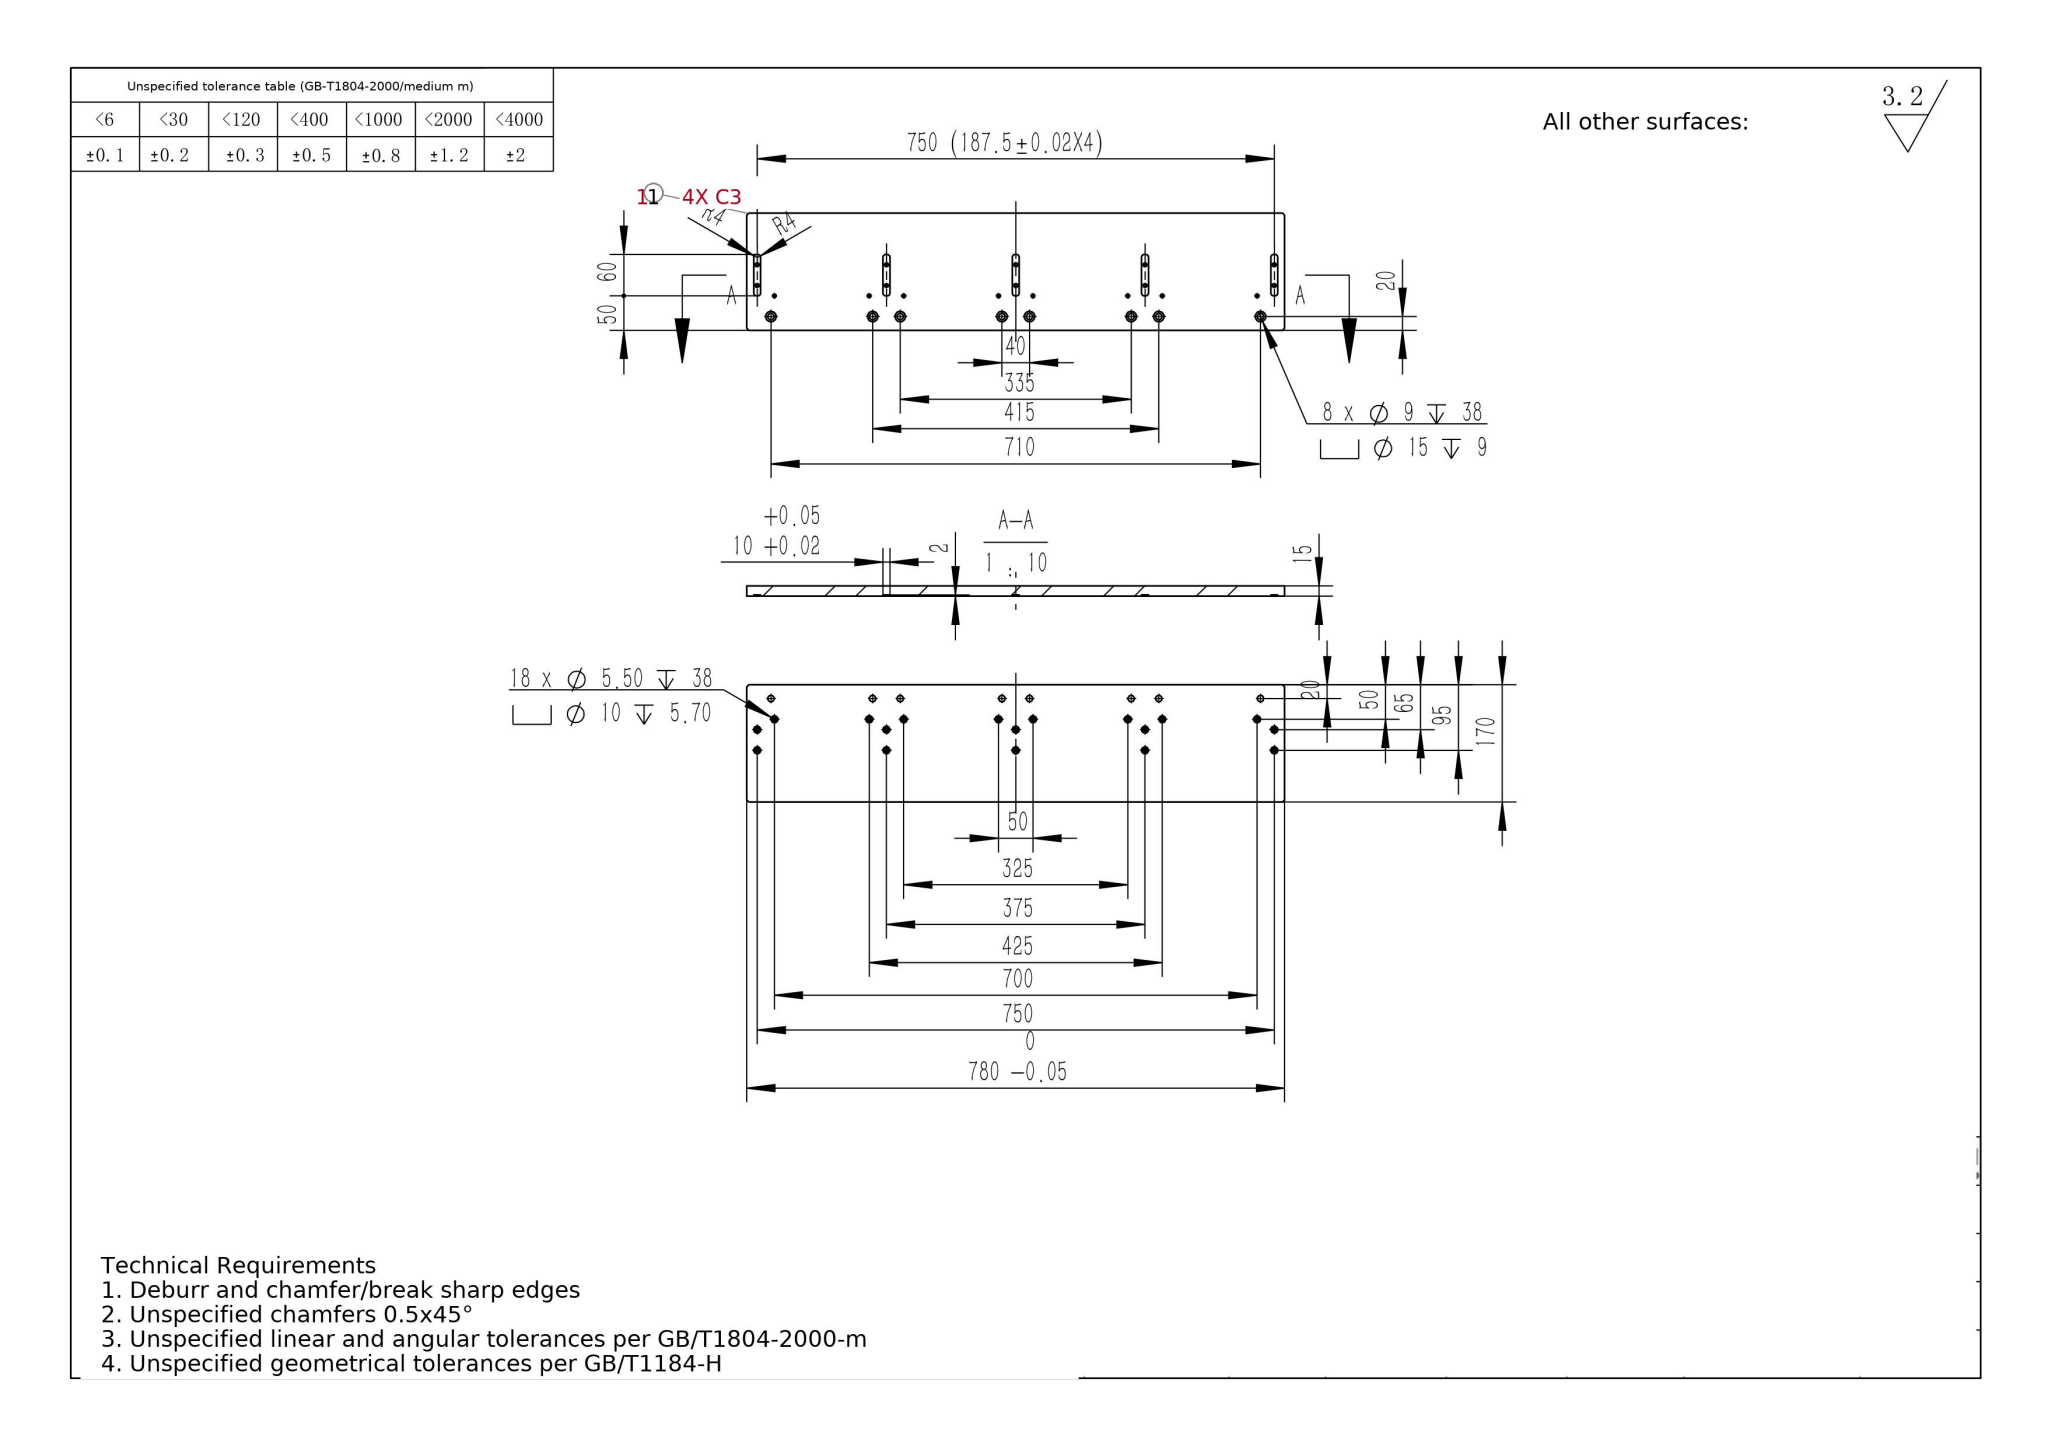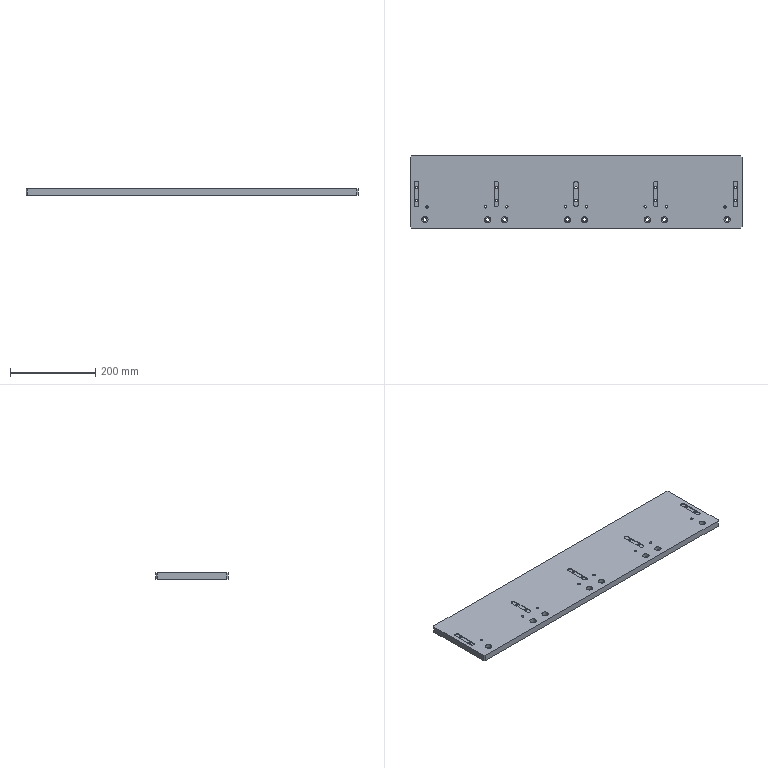Part | SolidWorks | mm | 1 solid | 185 faces | box 780 x 170 x 15 mm | volume 1955530 mm3 | cylinder 124 | plane 61 | commonest cylinder face diameters 10 x36 5.5 x36 8 x20 15 x16 9 x16
build123d program:
from build123d import *

# Parameters (mm, degrees)
SKETCH1_W                                         = 780
SKETCH1_H                                         = 170
BOSS_EXTRUDE1_DEPTH                               = 7.5
SKETCH2_W                                         = 10
SKETCH2_H                                         = 60
CUT_EXTRUDE1_DEPTH                                = 2
HOLE_SIZE_ACCORDING_TO_HEXAGON_SOCKET_D           = 9
HOLE_SIZE_ACCORDING_TO_HEXAGON_SOCKET_DEPTH       = 38
HOLE_SIZE_ACCORDING_TO_HEXAGON_SOCKET_CBORE_D     = 15
HOLE_SIZE_ACCORDING_TO_HEXAGON_SOCKET_CBORE_DEPTH = 9
HOLE_SIZE_ACCORDING_TO_HEXAGON_SOCKET_TIP         = 2.704
HOLE_SIZE_ACCORDING_TO_HEXAGON_SO_2_D             = 5.5
HOLE_SIZE_ACCORDING_TO_HEXAGON_SO_2_DEPTH         = 38
HOLE_SIZE_ACCORDING_TO_HEXAGON_SO_2_CBORE_D       = 10
HOLE_SIZE_ACCORDING_TO_HEXAGON_SO_2_CBORE_DEPTH   = 5.7
HOLE_SIZE_ACCORDING_TO_HEXAGON_SO_2_TIP           = 1.652
FILLET1_R                                         = 4
CHAMFER1_SIZE                                     = 3
HOLE_SIZE_ACCORDING_TO_HEXAGON_SO_3_D             = 5.5
HOLE_SIZE_ACCORDING_TO_HEXAGON_SO_3_DEPTH         = 38
HOLE_SIZE_ACCORDING_TO_HEXAGON_SO_3_CBORE_D       = 10
HOLE_SIZE_ACCORDING_TO_HEXAGON_SO_3_CBORE_DEPTH   = 5.7
HOLE_SIZE_ACCORDING_TO_HEXAGON_SO_3_TIP           = 1.652


with BuildPart() as part:
    # Sketch1 → Boss-Extrude1 (new, symmetric)
    with BuildSketch(Plane.XY):
        Rectangle(SKETCH1_W, SKETCH1_H)
    extrude(amount=BOSS_EXTRUDE1_DEPTH, both=True)

    # Sketch2 → Cut-Extrude1 (cut)
    with BuildSketch(Plane.XY.offset(7.5)):
        with Locations((-375, -5)):
            Rectangle(SKETCH2_W, SKETCH2_H)
        with Locations((-187.5, -5)):
            Rectangle(SKETCH2_W, SKETCH2_H)
        with Locations((187.5, -5)):
            Rectangle(SKETCH2_W, SKETCH2_H)
        with Locations((375, -5)):
            Rectangle(SKETCH2_W, SKETCH2_H)
        with Locations((0, -5)):
            Rectangle(SKETCH2_W, SKETCH2_H)
    extrude(amount=-CUT_EXTRUDE1_DEPTH, mode=Mode.SUBTRACT)

    # Hole Size _ according to_ Hexagon Socket
    with Locations(Plane.XY.offset(7.5)):
        with Locations((-355, -65), (-207.5, -65), (-167.5, -65), (167.5, -65), (207.5, -65), (355, -65), (-20, -65), (20, -65)):
            CounterBoreHole(HOLE_SIZE_ACCORDING_TO_HEXAGON_SOCKET_D / 2, HOLE_SIZE_ACCORDING_TO_HEXAGON_SOCKET_CBORE_D / 2, HOLE_SIZE_ACCORDING_TO_HEXAGON_SOCKET_CBORE_DEPTH, depth=HOLE_SIZE_ACCORDING_TO_HEXAGON_SOCKET_DEPTH)
            with Locations((0, 0, -(HOLE_SIZE_ACCORDING_TO_HEXAGON_SOCKET_DEPTH + HOLE_SIZE_ACCORDING_TO_HEXAGON_SOCKET_TIP / 2))):  # 118° drill point
                Cone(0, HOLE_SIZE_ACCORDING_TO_HEXAGON_SOCKET_D / 2, HOLE_SIZE_ACCORDING_TO_HEXAGON_SOCKET_TIP, mode=Mode.SUBTRACT)

    # Hole Size _ according to_ Hexagon So 2
    with Locations(Plane(origin=(0, 0, -7.5), x_dir=(-1, 0, 0), z_dir=(0, 0, -1))):
        with Locations((375, 10), (375, -20), (187.5, 10), (187.5, -20), (0, 10), (0, -20), (-187.5, -20), (-187.5, 10), (-375, -20), (-375, 10)):
            CounterBoreHole(HOLE_SIZE_ACCORDING_TO_HEXAGON_SO_2_D / 2, HOLE_SIZE_ACCORDING_TO_HEXAGON_SO_2_CBORE_D / 2, HOLE_SIZE_ACCORDING_TO_HEXAGON_SO_2_CBORE_DEPTH, depth=HOLE_SIZE_ACCORDING_TO_HEXAGON_SO_2_DEPTH)
            with Locations((0, 0, -(HOLE_SIZE_ACCORDING_TO_HEXAGON_SO_2_DEPTH + HOLE_SIZE_ACCORDING_TO_HEXAGON_SO_2_TIP / 2))):  # 118° drill point
                Cone(0, HOLE_SIZE_ACCORDING_TO_HEXAGON_SO_2_D / 2, HOLE_SIZE_ACCORDING_TO_HEXAGON_SO_2_TIP, mode=Mode.SUBTRACT)

    # Fillet1
    fillet1_edges = [part.edges().sort_by_distance(p)[0] for p in [
        (-380, -35, 6.5),
        (-380, 25, 6.5),
        (-370, 25, 6.5),
        (-370, -35, 6.5),
        (5, 25, 6.5),
        (5, -35, 6.5),
        (-5, -35, 6.5),
        (-5, 25, 6.5),
        (370, -35, 6.5),
        (370, 25, 6.5),
        (380, 25, 6.5),
        (380, -35, 6.5),
        (182.5, -35, 6.5),
        (182.5, 25, 6.5),
        (192.5, 25, 6.5),
        (192.5, -35, 6.5),
        (-192.5, -35, 6.5),
        (-192.5, 25, 6.5),
        (-182.5, 25, 6.5),
        (-182.5, -35, 6.5),
    ]]
    fillet(fillet1_edges, radius=FILLET1_R)

    # Chamfer1
    chamfer1_edges = [part.edges().sort_by_distance(p)[0] for p in [
        (390, -85, 0),
        (-390, -85, 0),
        (-390, 85, 0),
        (390, 85, 0),
    ]]
    chamfer(chamfer1_edges, length=CHAMFER1_SIZE)

    # Hole Size _ according to_ Hexagon So 3
    with Locations(Plane(origin=(0, 0, -7.5), x_dir=(-1, 0, 0), z_dir=(0, 0, -1))):
        with Locations((-350, -35), (-212.5, -35), (-162.5, -35), (-25, -35), (25, -35), (162.5, -35), (212.5, -35), (350, -35)):
            CounterBoreHole(HOLE_SIZE_ACCORDING_TO_HEXAGON_SO_3_D / 2, HOLE_SIZE_ACCORDING_TO_HEXAGON_SO_3_CBORE_D / 2, HOLE_SIZE_ACCORDING_TO_HEXAGON_SO_3_CBORE_DEPTH, depth=HOLE_SIZE_ACCORDING_TO_HEXAGON_SO_3_DEPTH)
            with Locations((0, 0, -(HOLE_SIZE_ACCORDING_TO_HEXAGON_SO_3_DEPTH + HOLE_SIZE_ACCORDING_TO_HEXAGON_SO_3_TIP / 2))):  # 118° drill point
                Cone(0, HOLE_SIZE_ACCORDING_TO_HEXAGON_SO_3_D / 2, HOLE_SIZE_ACCORDING_TO_HEXAGON_SO_3_TIP, mode=Mode.SUBTRACT)


solid = part.part